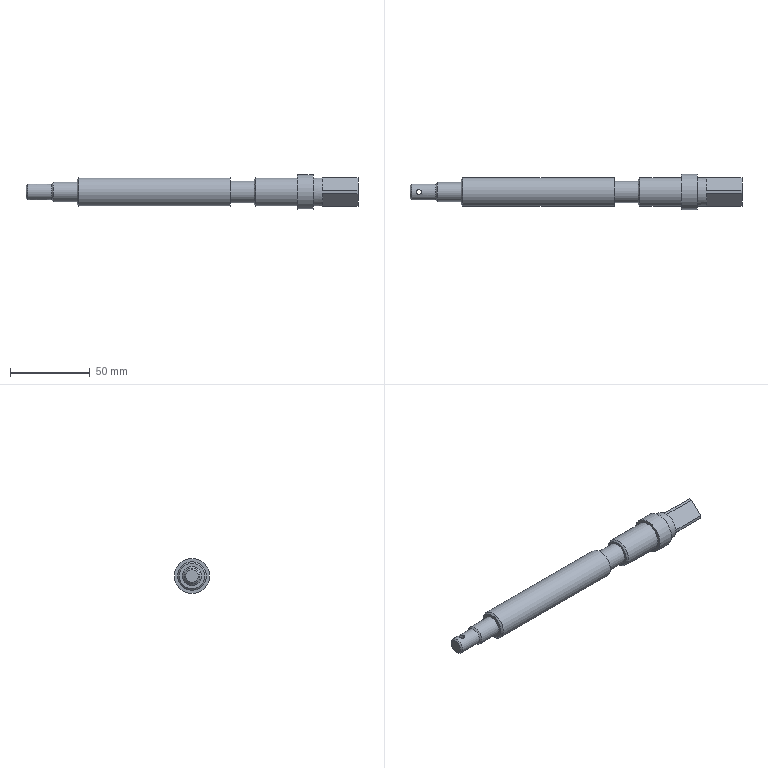Component | NX | 6 | 1 solid | 27 faces | volume 45918 mm3 | plane 15 | cylinder 8 | cone 4 | commonest cylinder face diameters 18 x3 10 x1 22 x1 13.5 x1 12 x1 3.1 x1